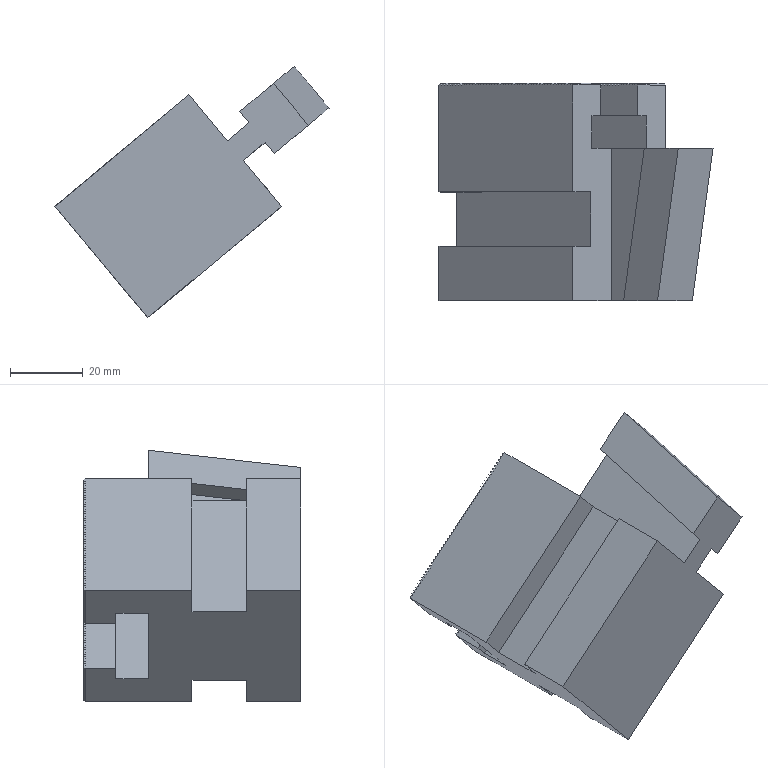Component | SolidWorks | K51-2_K51-2-1 | 1 solid | 220 faces | volume 97751 mm3 | plane 220